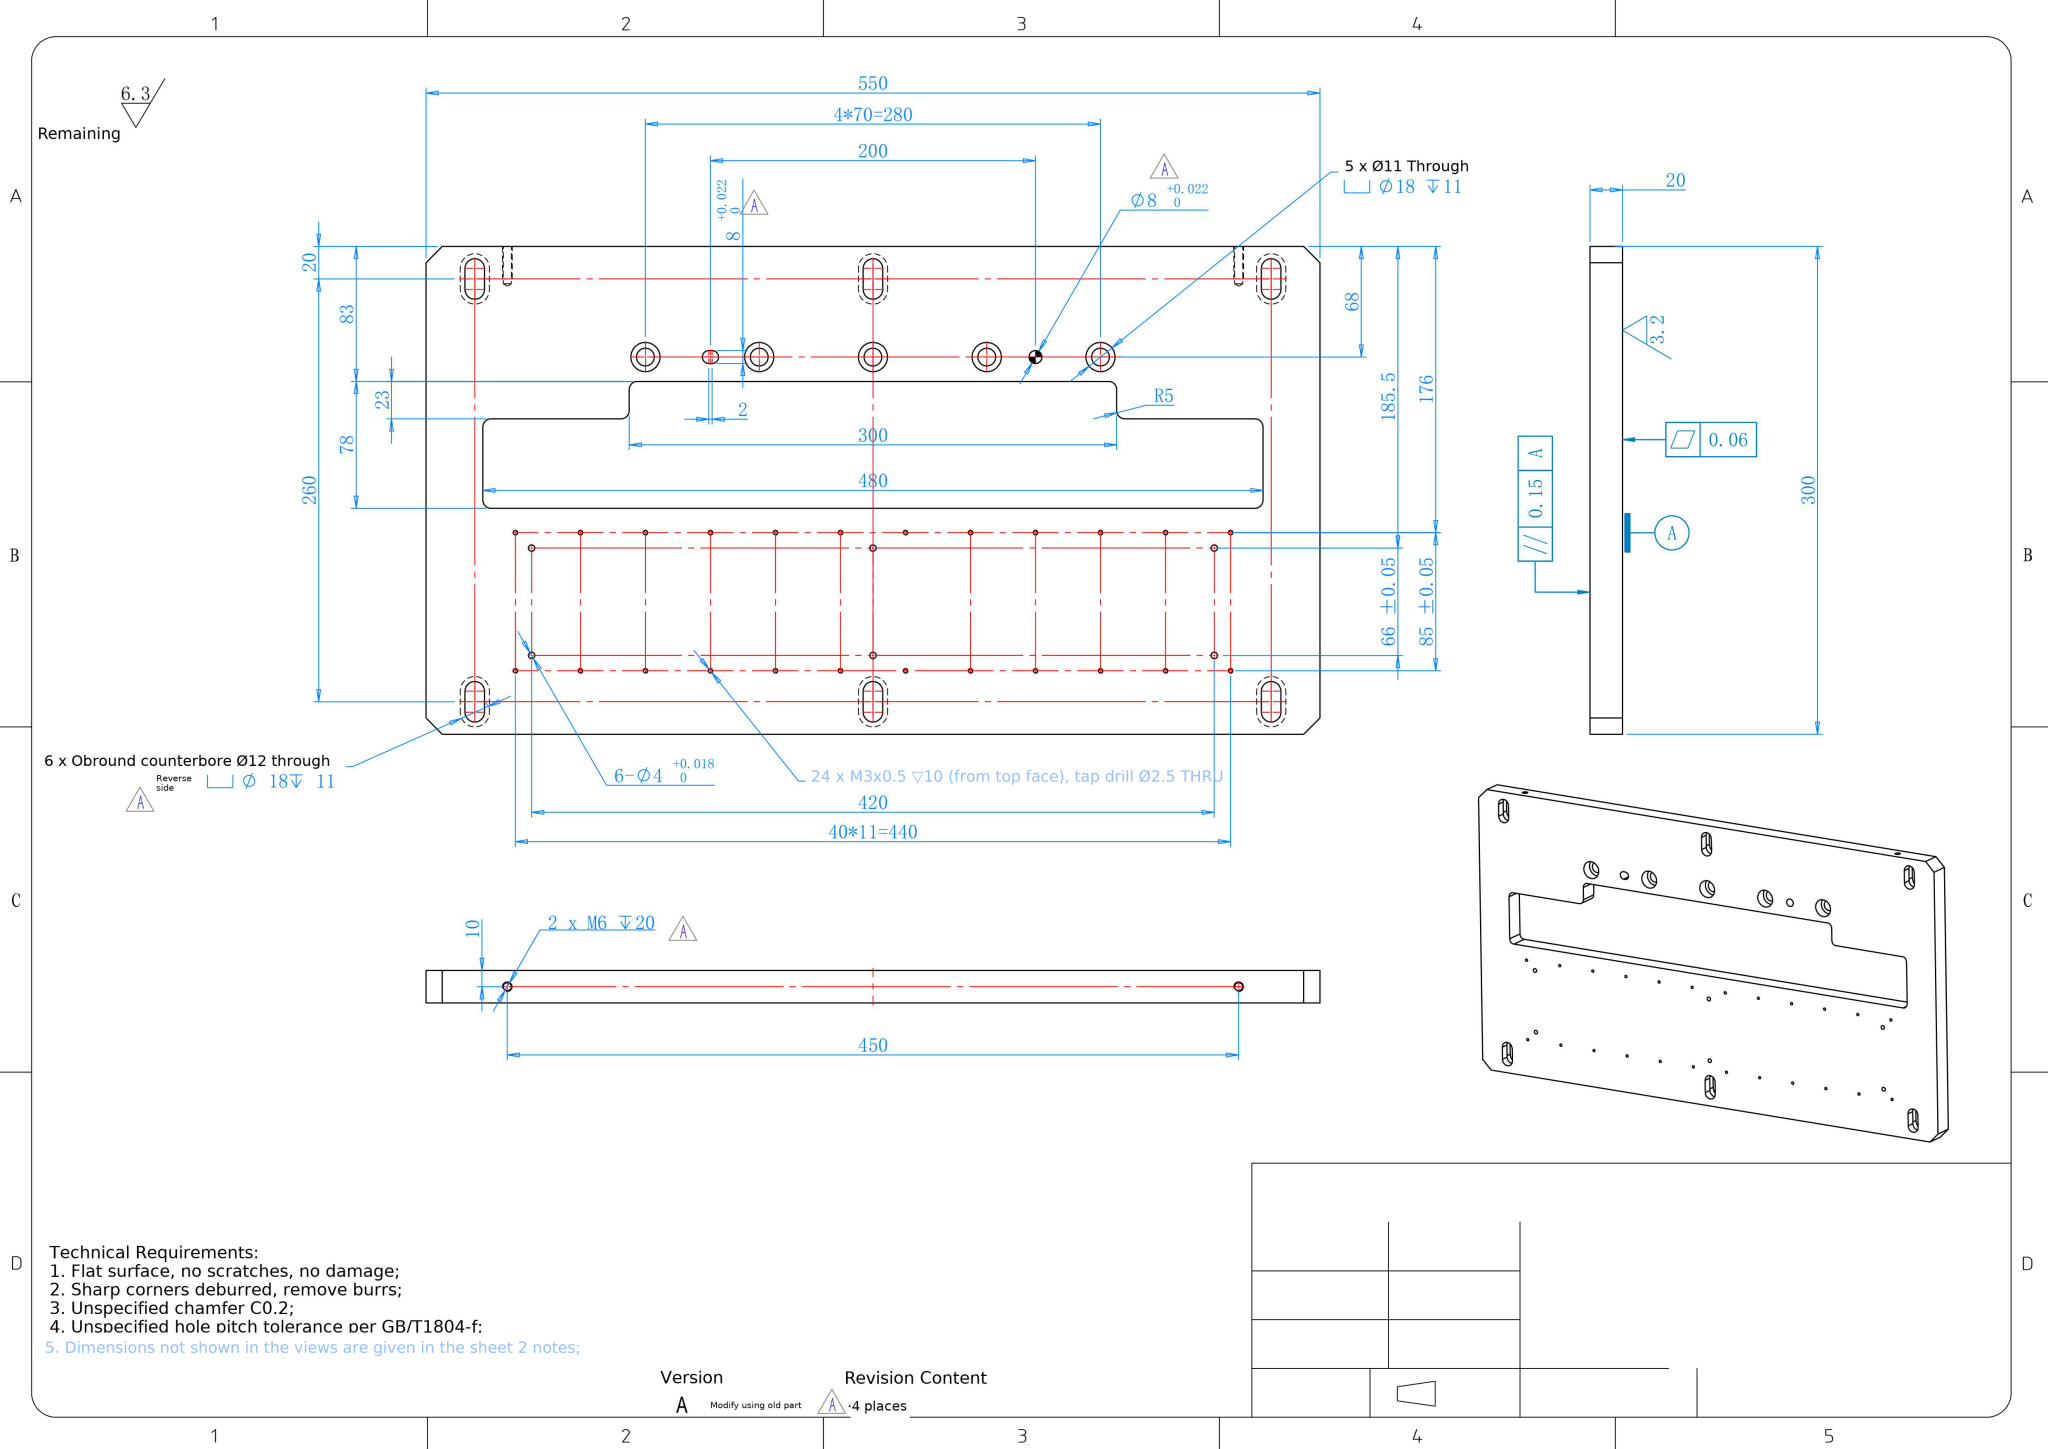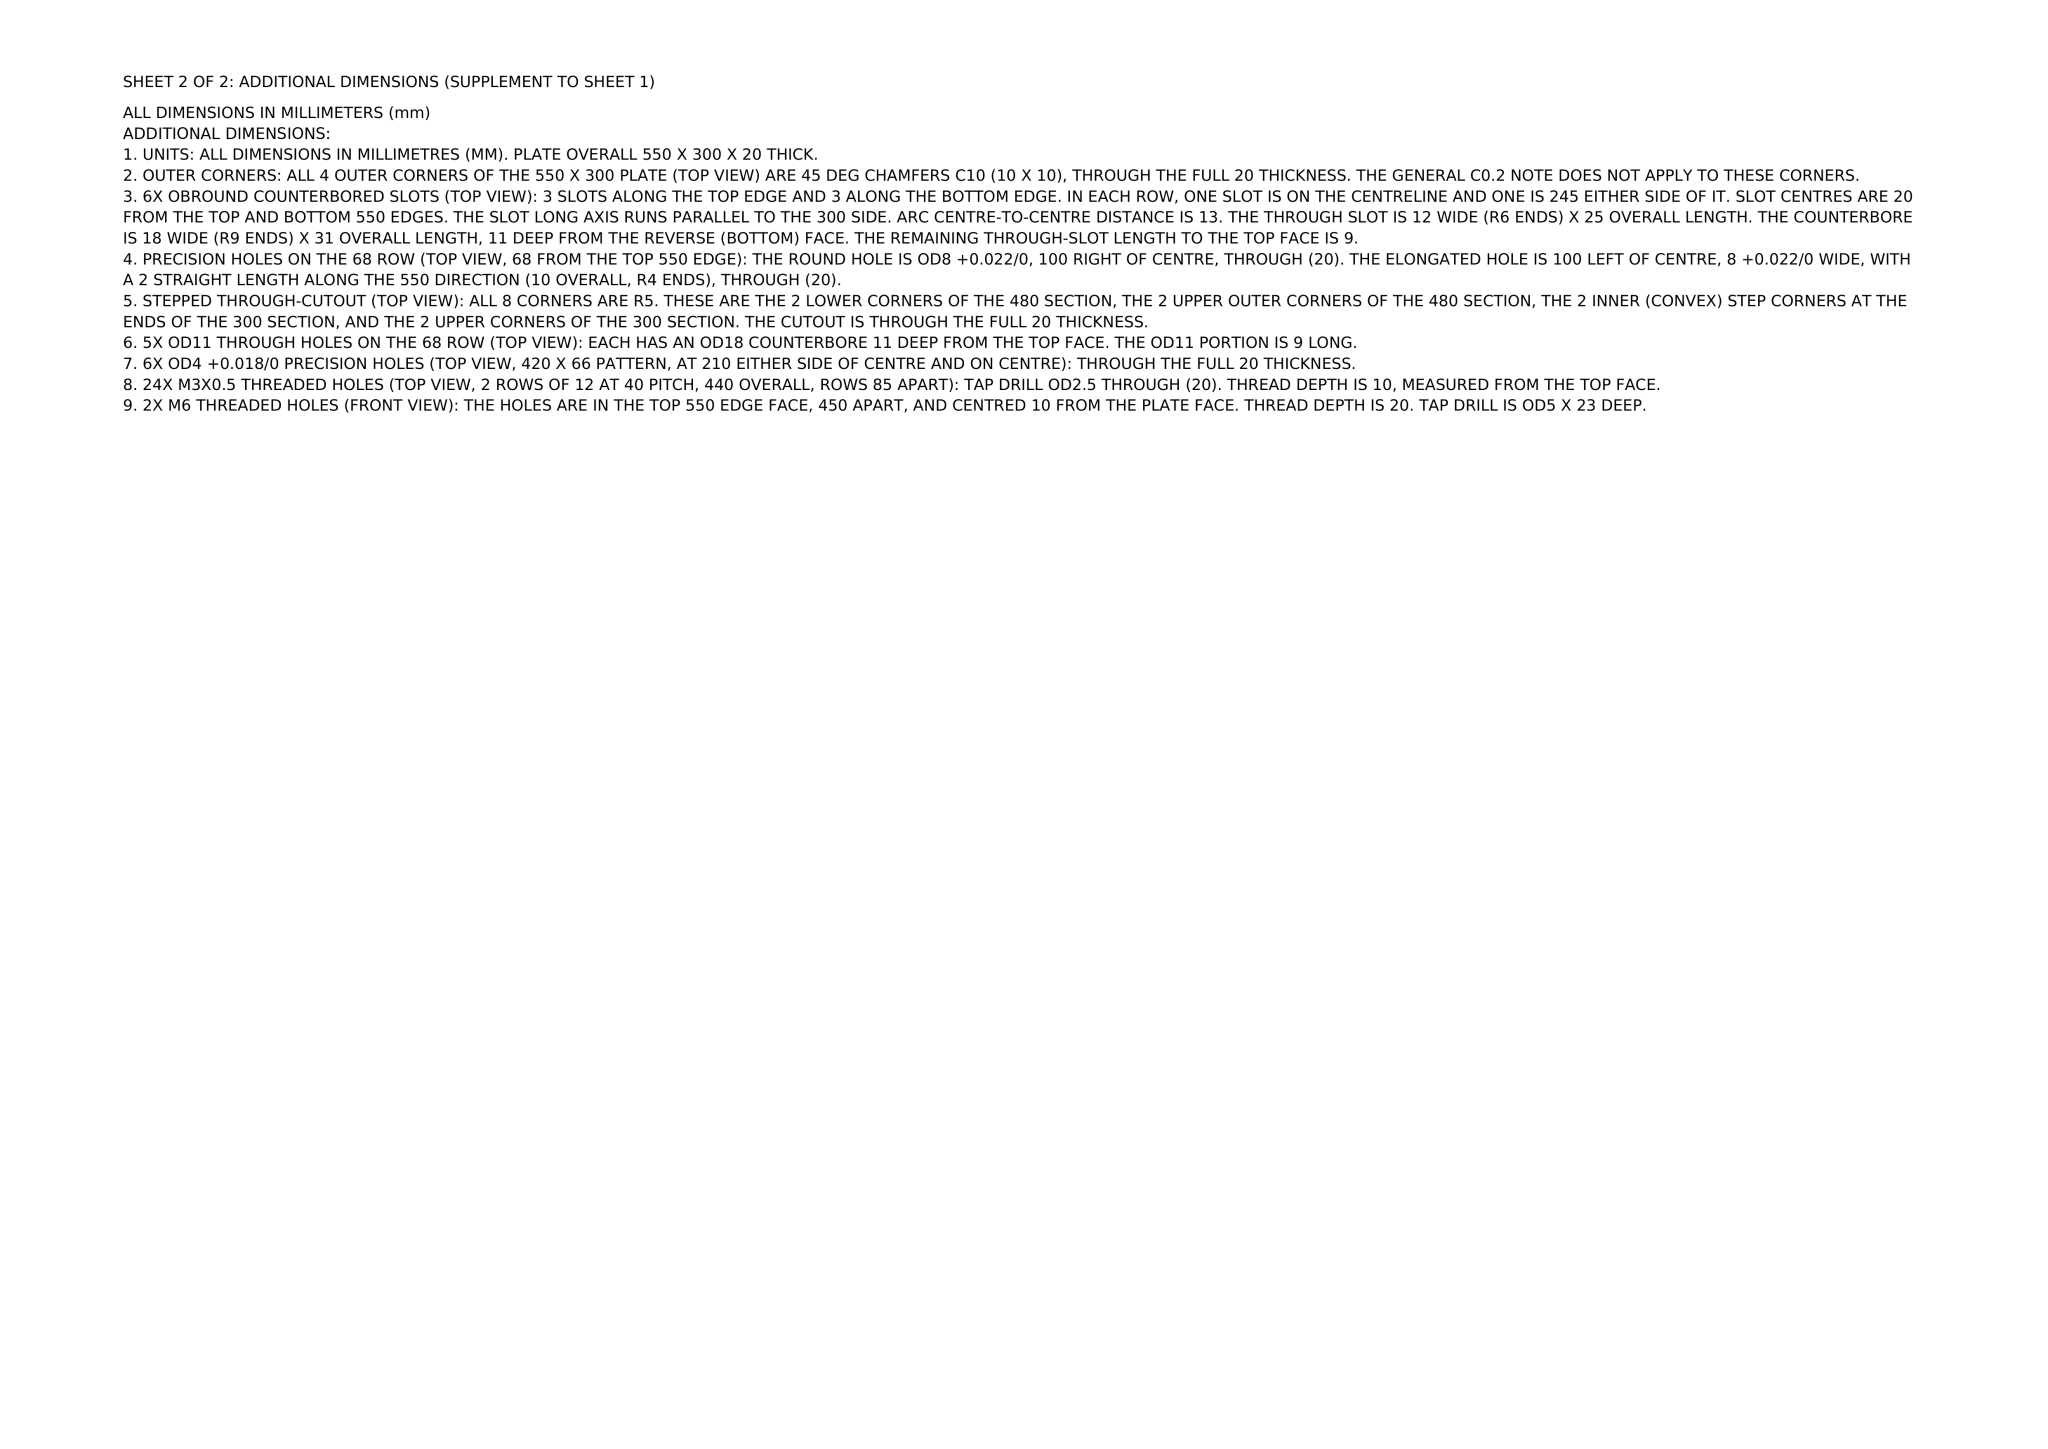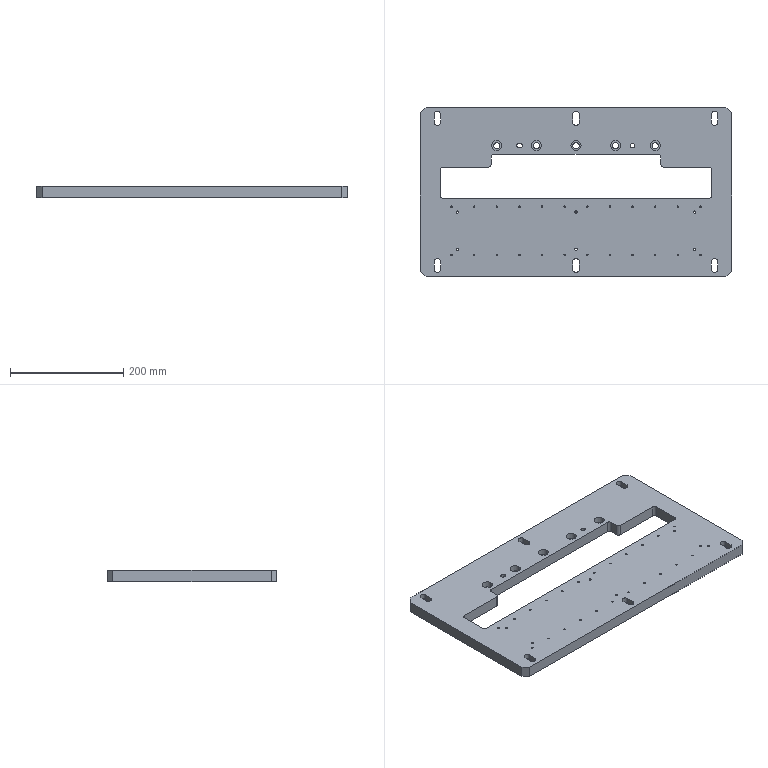Part | NX | mm | 1 solid | 180 faces | box 550 x 300 x 20 mm | volume 2558269 mm3 | cylinder 121 | plane 55 | cone 4 | commonest cylinder face diameters 2.5 x48 18 x22 4 x12 12 x12 11 x10 10 x8 8 x5 5 x4